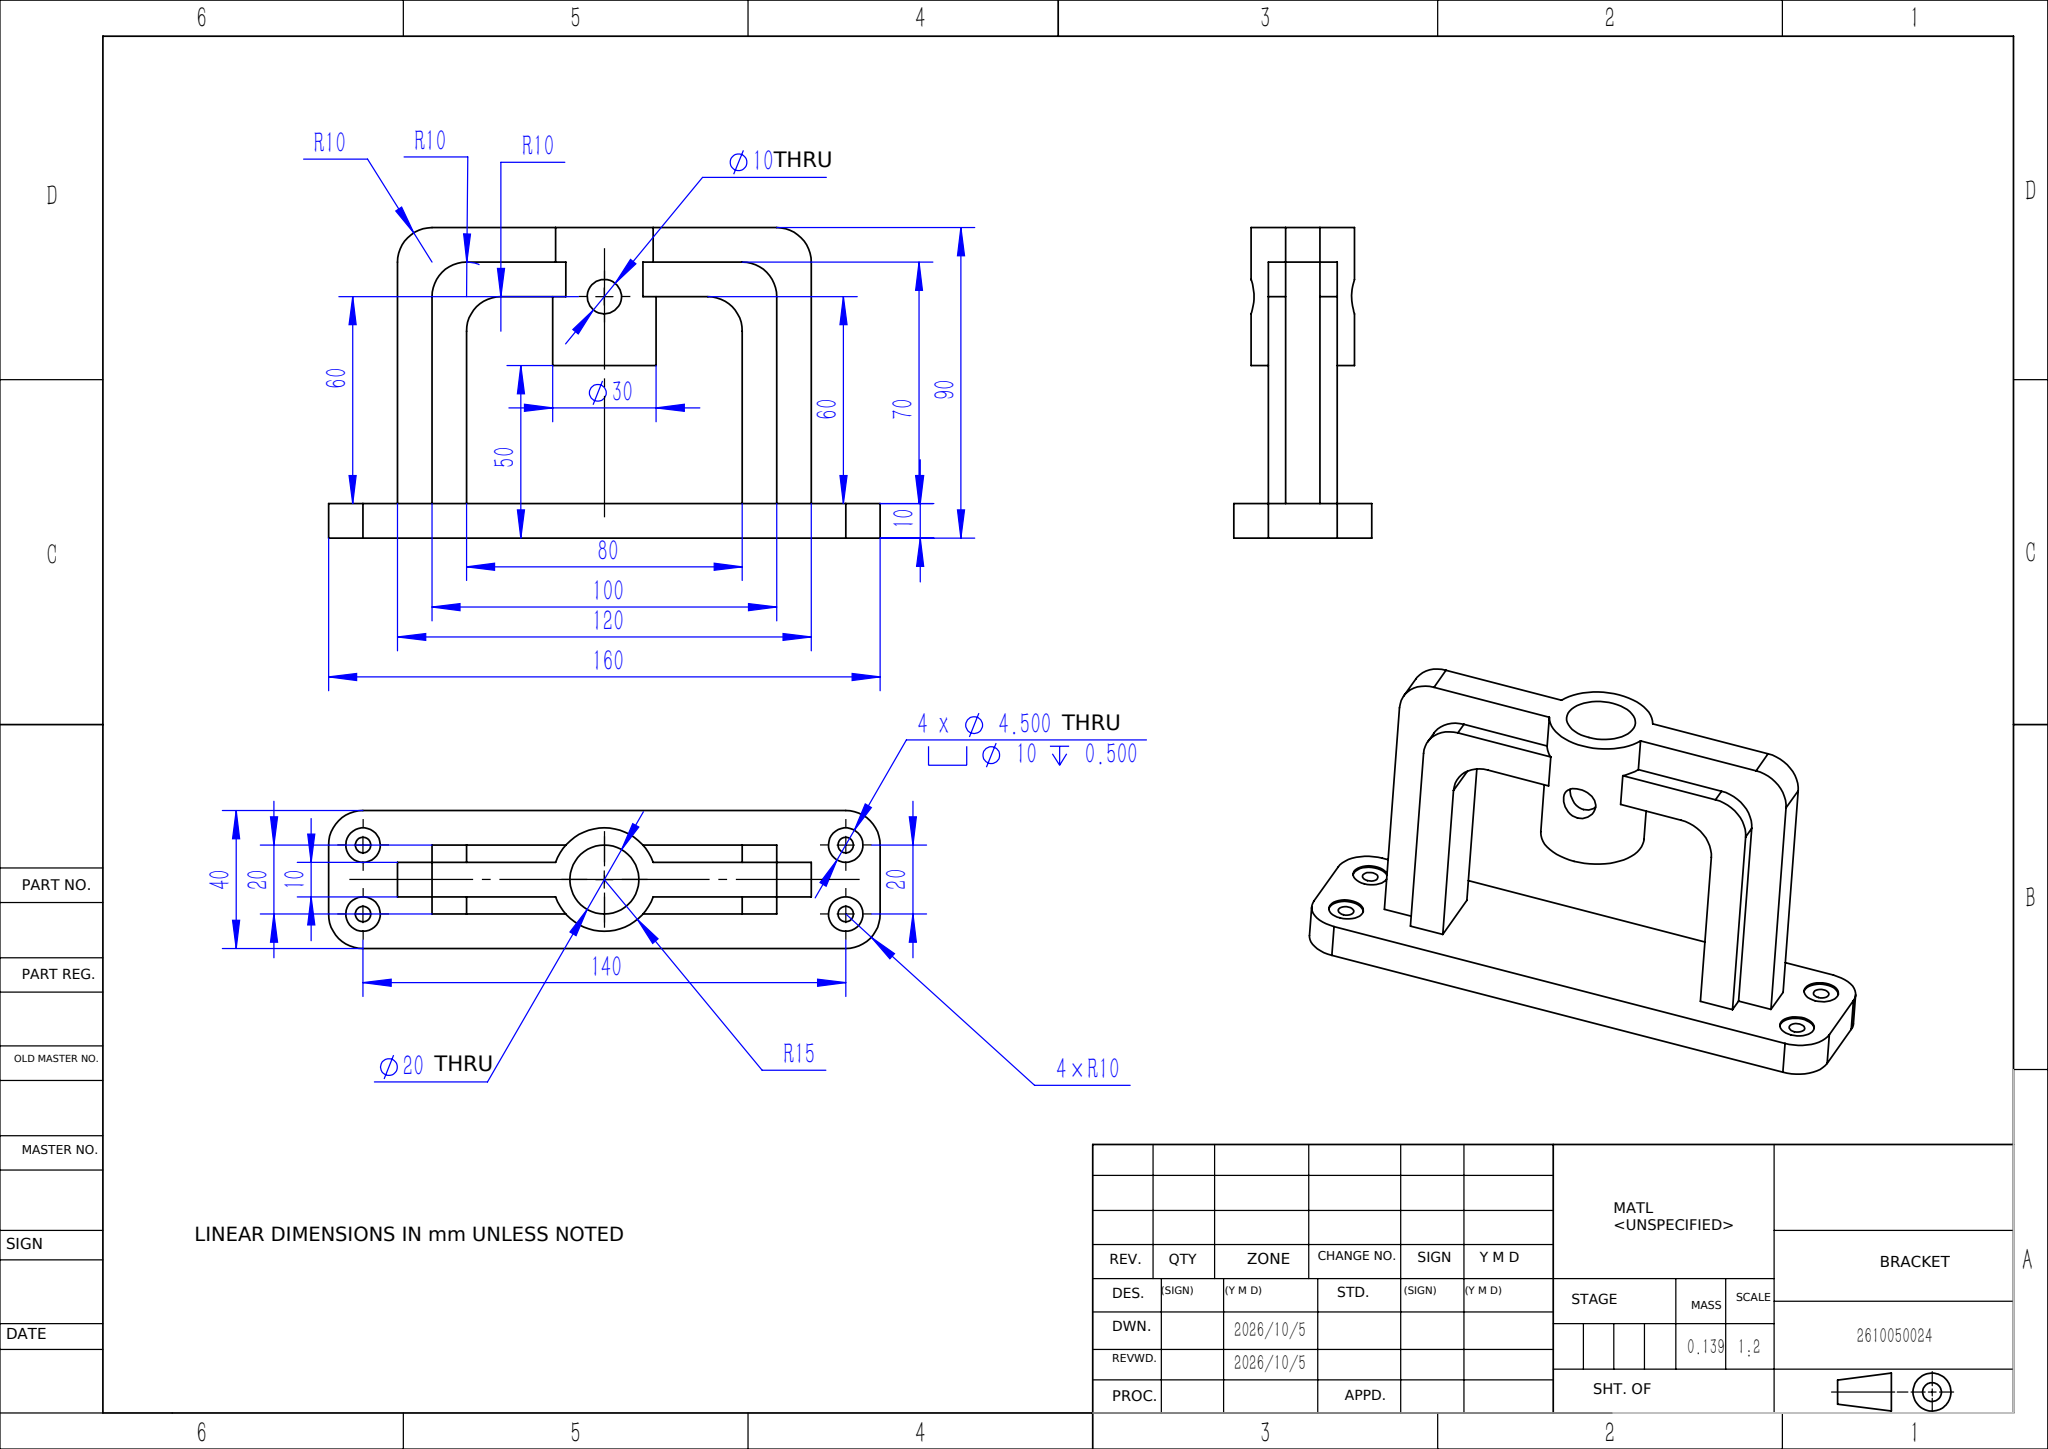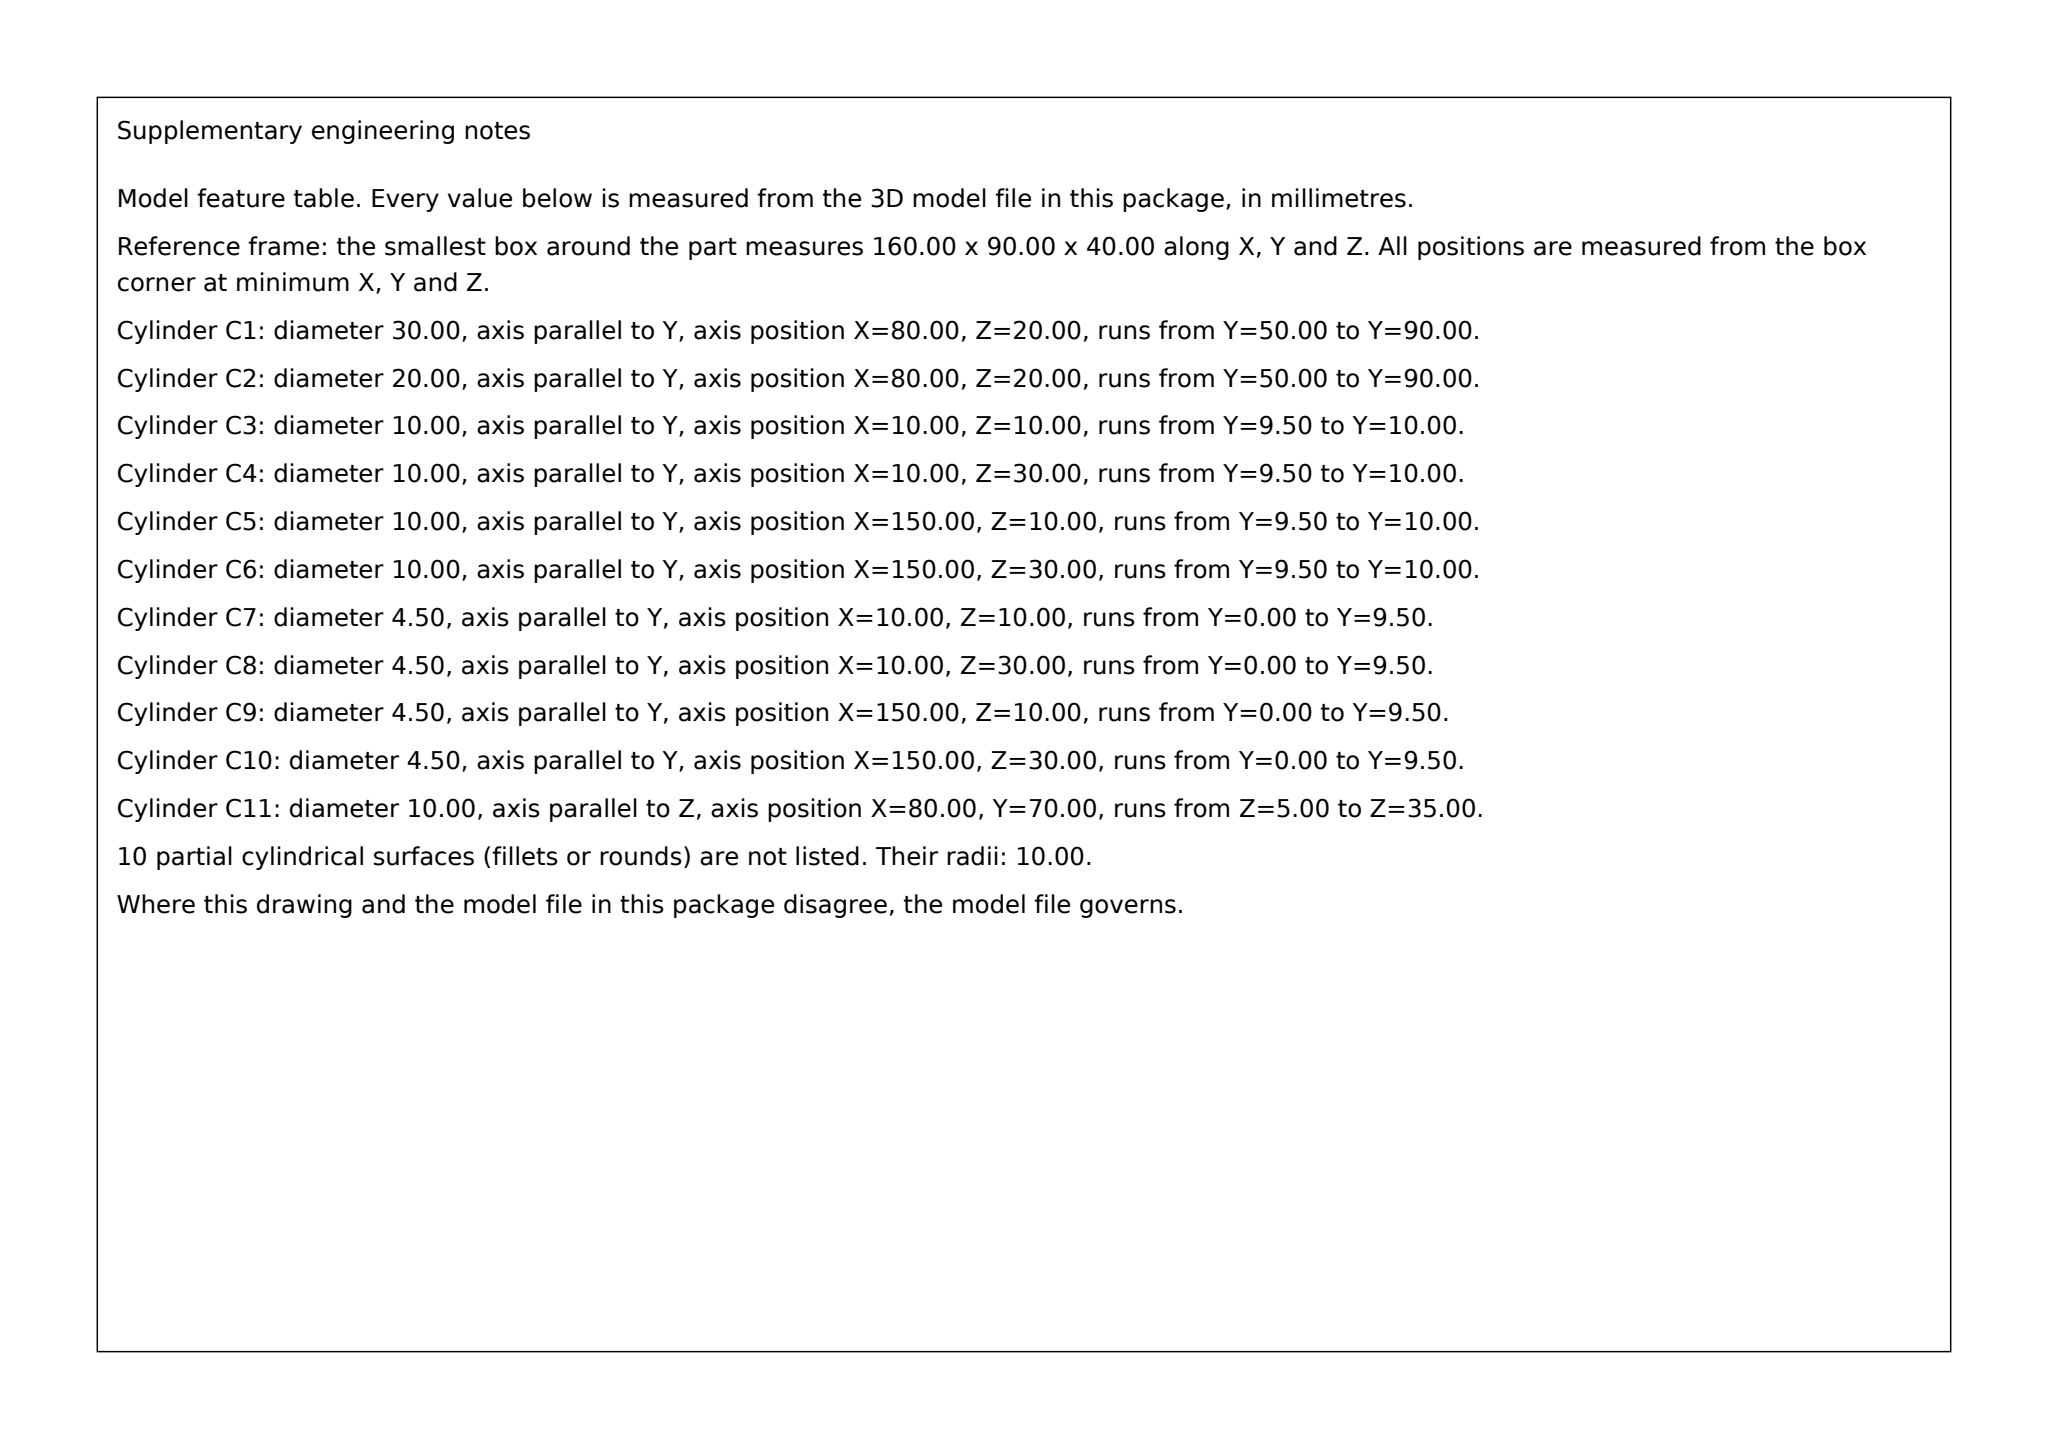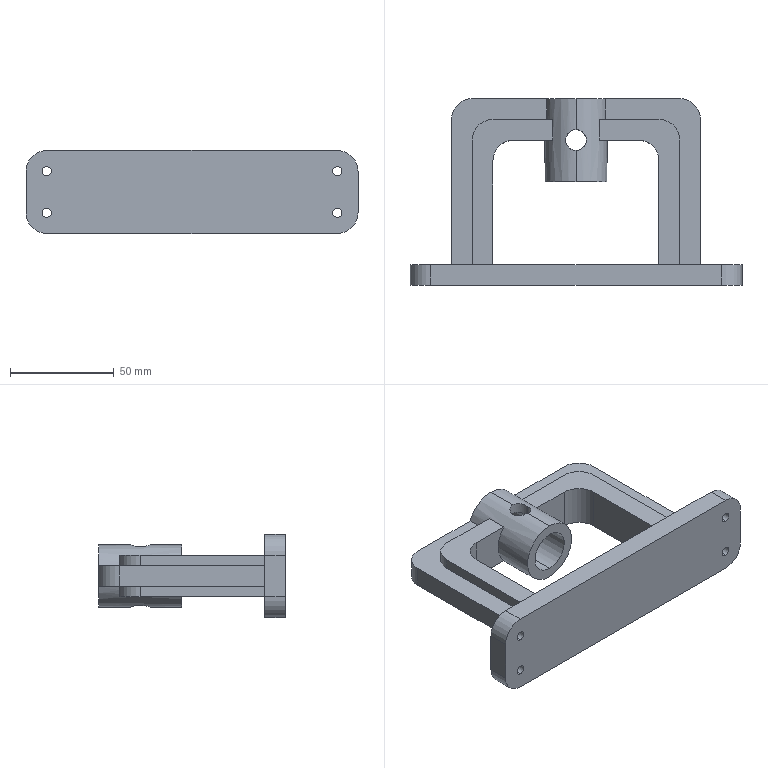Part | SolidWorks | mm | 1 solid | 70 faces | box 160 x 90 x 40 mm | volume 138822 mm3 | cylinder 36 | plane 34 | commonest cylinder face diameters 20 x14 10 x12 4.5 x8 30 x2
build123d program:
from build123d import *

# Parameters (mm, degrees)
BOSS_EXTRUDE1_DEPTH                                 = 5
BOSS_EXTRUDE2_DEPTH                                 = 10
SKETCH3_R                                           = 15
BOSS_EXTRUDE3_DEPTH                                 = 40
SKETCH4_R                                           = 10
CUT_EXTRUDE1_DEPTH                                  = 102.119
SKETCH5_W                                           = 160
SKETCH5_H                                           = 40
BOSS_EXTRUDE4_DEPTH                                 = 10
FILLET1_R                                           = 10
CYLINDRICAL_COUNTERSUNK_HOLE_FOR_M4_HEX_D           = 4.5
CYLINDRICAL_COUNTERSUNK_HOLE_FOR_M4_HEX_CBORE_D     = 10
CYLINDRICAL_COUNTERSUNK_HOLE_FOR_M4_HEX_CBORE_DEPTH = 0.5
CUT_EXTRUDE2_DEPTH                                  = 115.891
CUT_EXTRUDE2_DEPTH_BACK                             = 115.891
SKETCH9_R                                           = 5


with BuildPart() as part:
    # Sketch1 → Boss-Extrude1 (new, symmetric)
    with BuildSketch(Plane.XY):
        with BuildLine():
            Line((-40, 0), (-40, 50))
            ThreePointArc((-40, 50), (-37.071, 57.071), (-30, 60))
            Line((-30, 60), (30, 60))
            ThreePointArc((30, 60), (37.071, 57.071), (40, 50))
            Line((40, 50), (40, 0))
            Line((40, 0), (60, 0))
            Line((60, 0), (60, 70))
            ThreePointArc((60, 70), (57.071, 77.071), (50, 80))
            Line((50, 80), (-50, 80))
            ThreePointArc((-50, 80), (-57.071, 77.071), (-60, 70))
            Line((-60, 70), (-60, 0))
            Line((-60, 0), (-40, 0))
        make_face()
    extrude(amount=BOSS_EXTRUDE1_DEPTH, both=True)

    # Sketch2 → Boss-Extrude2 (add, symmetric)
    with BuildSketch(Plane.XY):
        with BuildLine():
            Line((-40, 0), (-40, 50))
            ThreePointArc((-40, 50), (-37.071, 57.071), (-30, 60))
            Line((-30, 60), (30, 60))
            ThreePointArc((30, 60), (37.071, 57.071), (40, 50))
            Line((40, 50), (40, 0))
            Line((40, 0), (50, 0))
            Line((50, 0), (50, 60))
            ThreePointArc((50, 60), (47.071, 67.071), (40, 70))
            Line((40, 70), (-40, 70))
            ThreePointArc((-40, 70), (-47.071, 67.071), (-50, 60))
            Line((-50, 60), (-50, 0))
            Line((-50, 0), (-40, 0))
        make_face()
    extrude(amount=BOSS_EXTRUDE2_DEPTH, both=True)

    # Sketch3 → Boss-Extrude3 (add)
    with BuildSketch(Plane(origin=(0, 80, 0), x_dir=(1, 0, 0), z_dir=(0, 1, 0))):
        with Locations(Location((0, 0, 0), (0, 0, 270))):
            Circle(SKETCH3_R)
    extrude(amount=-BOSS_EXTRUDE3_DEPTH)

    # Sketch4 → Cut-Extrude1 (cut, through all)
    with BuildSketch(Plane(origin=(0, 80, 0), x_dir=(1, 0, 0), z_dir=(0, 1, 0))):
        with Locations(Location((0, 0, 0), (0, 0, 270))):
            Circle(SKETCH4_R)
    extrude(amount=-CUT_EXTRUDE1_DEPTH, mode=Mode.SUBTRACT)

    # Sketch5 → Boss-Extrude4 (add)
    with BuildSketch(Plane.XZ):
        Rectangle(SKETCH5_W, SKETCH5_H)
    extrude(amount=BOSS_EXTRUDE4_DEPTH)

    # Fillet1
    fillet1_edges = [part.edges().sort_by_distance(p)[0] for p in [
        (80, -5, -20),
        (80, -5, 20),
        (-80, -5, 20),
        (-80, -5, -20),
    ]]
    fillet(fillet1_edges, radius=FILLET1_R)

    # Cylindrical Countersunk Hole for M4 Hex (through all)
    with Locations(Plane(origin=(0, 0, 0), x_dir=(1, 0, 0), z_dir=(0, 1, 0))):
        with Locations((-70, 10), (-70, -10), (70, 10), (70, -10)):
            CounterBoreHole(CYLINDRICAL_COUNTERSUNK_HOLE_FOR_M4_HEX_D / 2, CYLINDRICAL_COUNTERSUNK_HOLE_FOR_M4_HEX_CBORE_D / 2, CYLINDRICAL_COUNTERSUNK_HOLE_FOR_M4_HEX_CBORE_DEPTH)

    # Sketch9 → Cut-Extrude2 (cut, two sides: drawn at the far end of the back side and taken through both)
    with BuildSketch(Plane.XY.offset(-CUT_EXTRUDE2_DEPTH_BACK)):
        with Locations((0, 60)):
            Circle(SKETCH9_R)
    extrude(amount=CUT_EXTRUDE2_DEPTH + CUT_EXTRUDE2_DEPTH_BACK, mode=Mode.SUBTRACT)


solid = part.part